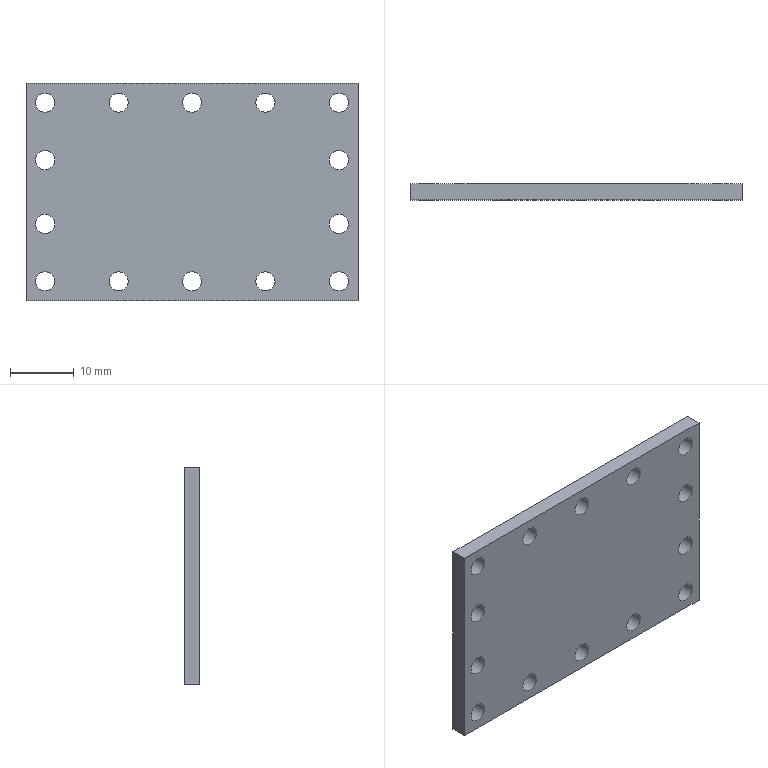Component | NX | EXT_END_PLATE | 1 solid | 29 faces | volume 3756 mm3 | cylinder 18 | plane 11 | commonest cylinder face diameters 3 x14 4 x4